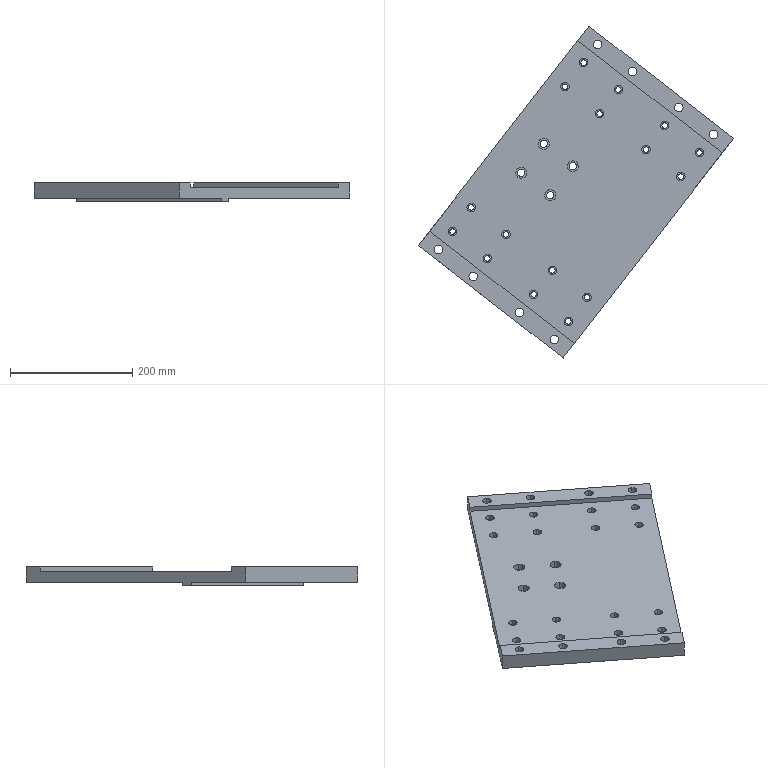Component | SolidWorks | 0803_205_Plate-1 | 1 solid | 154 faces | box 515.98 x 543.38 x 30 mm | volume 2399297 mm3 | cylinder 112 | plane 42 | commonest cylinder face diameters 14 x48 9 x32 20 x16 18 x8 12 x8
build123d program:
from build123d import *

# Parameters (mm, degrees)
SKETCH1_W                                        = 455
SKETCH1_H                                        = 300
BOSS_EXTRUDE1_DEPTH                              = 30
SKETCH2_W                                        = 324
SKETCH2_H                                        = 300
SKETCH2_W_2                                      = 112.5
CUT_EXTRUDE1_DEPTH                               = 5
SKETCH3_W                                        = 395
SKETCH3_H                                        = 300
CUT_EXTRUDE2_DEPTH                               = 8
CBORE_FOR_M12_SOCKET_HEAD_CAP_SCREW1_D           = 14
CBORE_FOR_M12_SOCKET_HEAD_CAP_SCREW1_CBORE_D     = 20
CBORE_FOR_M12_SOCKET_HEAD_CAP_SCREW1_CBORE_DEPTH = 14
LPATTERN1_COUNT                                  = 2
LPATTERN1_PITCH                                  = 425
CBORE_FOR_M8_SOCKET_HEAD_CAP_SCREW1_D            = 9
CBORE_FOR_M8_SOCKET_HEAD_CAP_SCREW1_CBORE_D      = 14
CBORE_FOR_M8_SOCKET_HEAD_CAP_SCREW1_CBORE_DEPTH  = 9
LPATTERN2_COUNT                                  = 2
LPATTERN2_PITCH                                  = 300
LPATTERN2_COUNT_DIR2                             = 2
LPATTERN2_PITCH_DIR2                             = 168
CBORE_FOR_M10_SOCKET_HEAD_CAP_SCREW1_D           = 12
CBORE_FOR_M10_SOCKET_HEAD_CAP_SCREW1_CBORE_D     = 18
CBORE_FOR_M10_SOCKET_HEAD_CAP_SCREW1_CBORE_DEPTH = 11


with BuildPart() as part:
    # Sketch1 → Boss-Extrude1 (new body)
    with BuildSketch(Plane.XY):
        with Locations((-227.5, 150)):
            Rectangle(SKETCH1_W, SKETCH1_H)
    extrude(amount=-BOSS_EXTRUDE1_DEPTH)

    # Sketch2 → Cut-Extrude1 (cut)
    with BuildSketch(Plane(origin=(0, 0, -30), x_dir=(-1, 0, 0), z_dir=(0, 0, -1))):
        with Locations((162, 150)):
            Rectangle(SKETCH2_W, SKETCH2_H)
        with Locations((398.75, 150)):
            Rectangle(SKETCH2_W_2, SKETCH2_H)
    extrude(amount=-CUT_EXTRUDE1_DEPTH, mode=Mode.SUBTRACT)

    # Sketch3 → Cut-Extrude2 (cut)
    with BuildSketch(Plane.XY):
        with Locations((-227.5, 150)):
            Rectangle(SKETCH3_W, SKETCH3_H)
    extrude(amount=-CUT_EXTRUDE2_DEPTH, mode=Mode.SUBTRACT)

    # CBORE for M12 Socket Head Cap Screw1 (through all)
    with Locations(Plane(origin=(-5.933, 68.021, -25), x_dir=(1, 0, 0), z_dir=(0, 0, -1))):
        with Locations((-9.067, -201.979), (-9.067, -129.979), (-9.067, -33.979), (-9.067, 38.021)):
            cbore_for_m12_socket_head_cap_screw1 = CounterBoreHole(CBORE_FOR_M12_SOCKET_HEAD_CAP_SCREW1_D / 2, CBORE_FOR_M12_SOCKET_HEAD_CAP_SCREW1_CBORE_D / 2, CBORE_FOR_M12_SOCKET_HEAD_CAP_SCREW1_CBORE_DEPTH)

    # LPattern1: CBORE for M12 Socket Head Cap Screw1 ×2
    with Locations(*[(-i * LPATTERN1_PITCH, 0, 0) for i in range(1, LPATTERN1_COUNT)]):
        add(cbore_for_m12_socket_head_cap_screw1, mode=Mode.SUBTRACT)

    # CBORE for M8 Socket Head Cap Screw1 (through all)
    with Locations(Plane.XY.offset(-8)):
        with Locations((-52.5, 30), (-52.5, 102), (-102.5, 102), (-102.5, 30)):
            cbore_for_m8_socket_head_cap_screw1 = CounterBoreHole(CBORE_FOR_M8_SOCKET_HEAD_CAP_SCREW1_D / 2, CBORE_FOR_M8_SOCKET_HEAD_CAP_SCREW1_CBORE_D / 2, CBORE_FOR_M8_SOCKET_HEAD_CAP_SCREW1_CBORE_DEPTH)

    # LPattern2: CBORE for M8 Socket Head Cap Screw1 2 × 2
    with Locations(*[(-i * LPATTERN2_PITCH, j * LPATTERN2_PITCH_DIR2, 0) for i in range(LPATTERN2_COUNT) for j in range(LPATTERN2_COUNT_DIR2) if (i, j) != (0, 0)]):
        add(cbore_for_m8_socket_head_cap_screw1, mode=Mode.SUBTRACT)

    # CBORE for M10 Socket Head Cap Screw1 (through all)
    with Locations(Plane.XY.offset(-8)):
        with Locations((-197.5, 240), (-197.5, 180), (-257.5, 180), (-257.5, 240)):
            CounterBoreHole(CBORE_FOR_M10_SOCKET_HEAD_CAP_SCREW1_D / 2, CBORE_FOR_M10_SOCKET_HEAD_CAP_SCREW1_CBORE_D / 2, CBORE_FOR_M10_SOCKET_HEAD_CAP_SCREW1_CBORE_DEPTH)


solid = part.part

# Placed as in the assembly
solid = solid.moved(Location((409.235, 714.967, 381.411), (0, 0, 52.179)))